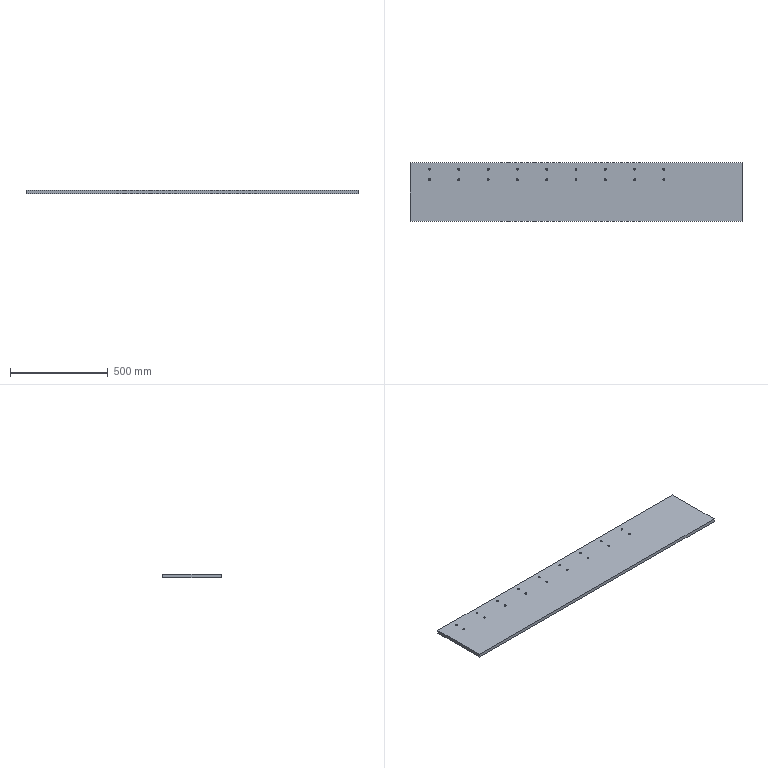Component | SolidWorks | X-AxisSlideMountingPlate-1 | 1 solid | 204 faces | box 1700 x 300 x 17 mm | volume 8657405 mm3 | cone 108 | cylinder 72 | plane 24 | commonest cylinder face diameters 5.5 x36 10 x36
build123d program:
from build123d import *

# Parameters (mm, degrees)
SKETCH1_W                                      = 1700
SKETCH1_H                                      = 300
BOSS_EXTRUDE1_DEPTH                            = 17
M5_HEX_SOCKET_HEAD_CAP_SCREW_CBORE1_AT_2_COUNT = 2
M5_HEX_SOCKET_HEAD_CAP_SCREW_CBORE1_AT_2_PITCH = 54
LPATTERN1_COUNT                                = 9
LPATTERN1_PITCH                                = 150


with BuildPart() as part:
    # Sketch1 → Boss-Extrude1 (new body)
    with BuildSketch(Plane.XY):
        Rectangle(SKETCH1_W, SKETCH1_H)
    extrude(amount=BOSS_EXTRUDE1_DEPTH)

    # Sketch3 → M5 Hex Socket Head Cap Screw CBORE1 (revolve, cut)
    with BuildSketch(Plane(origin=(450, 117, 17), x_dir=(0, -1, 0), z_dir=(1, 0, 0))):
        Polygon((0, 0), (0, 17), (2.775, 17), (2.75, 16.975), (2.75, 5.425), (2.775, 5.4), (5, 5.4), (5, 0.025), (5.025, 0), align=None)
    m5_hex_socket_head_cap_screw_cbore1 = revolve(axis=Axis((450, 117, 23.35), (0, 0, -1)), mode=Mode.SUBTRACT)

    # M5 Hex Socket Head Cap Screw CBORE1 at 2: M5 Hex Socket Head Cap Screw CBORE1 ×2
    with Locations(*[(0, -i * M5_HEX_SOCKET_HEAD_CAP_SCREW_CBORE1_AT_2_PITCH, 0) for i in range(1, M5_HEX_SOCKET_HEAD_CAP_SCREW_CBORE1_AT_2_COUNT)]):
        add(m5_hex_socket_head_cap_screw_cbore1, mode=Mode.SUBTRACT)

    # LPattern1: M5 Hex Socket Head Cap Screw CBORE1 ×9
    with Locations(*[(-i * LPATTERN1_PITCH, 0, 0) for i in range(1, LPATTERN1_COUNT)]):
        add(m5_hex_socket_head_cap_screw_cbore1, mode=Mode.SUBTRACT)

    # LPattern1 copy 1 sketch → LPattern1 copy 1 (revolve, cut)
    with BuildSketch(Plane(origin=(300, 63, 17), x_dir=(0, -1, 0), z_dir=(1, 0, 0))):
        Polygon((0, 0), (0, 17), (2.775, 17), (2.75, 16.975), (2.75, 5.425), (2.775, 5.4), (5, 5.4), (5, 0.025), (5.025, 0), align=None)
    revolve(axis=Axis((300, 63, 23.35), (0, 0, -1)), mode=Mode.SUBTRACT)

    # LPattern1 copy 2 sketch → LPattern1 copy 2 (revolve, cut)
    with BuildSketch(Plane(origin=(150, 63, 17), x_dir=(0, -1, 0), z_dir=(1, 0, 0))):
        Polygon((0, 0), (0, 17), (2.775, 17), (2.75, 16.975), (2.75, 5.425), (2.775, 5.4), (5, 5.4), (5, 0.025), (5.025, 0), align=None)
    revolve(axis=Axis((150, 63, 23.35), (0, 0, -1)), mode=Mode.SUBTRACT)

    # LPattern1 copy 3 sketch → LPattern1 copy 3 (revolve, cut)
    with BuildSketch(Plane(origin=(0, 63, 17), x_dir=(0, -1, 0), z_dir=(1, 0, 0))):
        Polygon((0, 0), (0, 17), (2.775, 17), (2.75, 16.975), (2.75, 5.425), (2.775, 5.4), (5, 5.4), (5, 0.025), (5.025, 0), align=None)
    revolve(axis=Axis((0, 63, 23.35), (0, 0, -1)), mode=Mode.SUBTRACT)

    # LPattern1 copy 4 sketch → LPattern1 copy 4 (revolve, cut)
    with BuildSketch(Plane(origin=(-150, 63, 17), x_dir=(0, -1, 0), z_dir=(1, 0, 0))):
        Polygon((0, 0), (0, 17), (2.775, 17), (2.75, 16.975), (2.75, 5.425), (2.775, 5.4), (5, 5.4), (5, 0.025), (5.025, 0), align=None)
    revolve(axis=Axis((-150, 63, 23.35), (0, 0, -1)), mode=Mode.SUBTRACT)

    # LPattern1 copy 5 sketch → LPattern1 copy 5 (revolve, cut)
    with BuildSketch(Plane(origin=(-300, 63, 17), x_dir=(0, -1, 0), z_dir=(1, 0, 0))):
        Polygon((0, 0), (0, 17), (2.775, 17), (2.75, 16.975), (2.75, 5.425), (2.775, 5.4), (5, 5.4), (5, 0.025), (5.025, 0), align=None)
    revolve(axis=Axis((-300, 63, 23.35), (0, 0, -1)), mode=Mode.SUBTRACT)

    # LPattern1 copy 6 sketch → LPattern1 copy 6 (revolve, cut)
    with BuildSketch(Plane(origin=(-450, 63, 17), x_dir=(0, -1, 0), z_dir=(1, 0, 0))):
        Polygon((0, 0), (0, 17), (2.775, 17), (2.75, 16.975), (2.75, 5.425), (2.775, 5.4), (5, 5.4), (5, 0.025), (5.025, 0), align=None)
    revolve(axis=Axis((-450, 63, 23.35), (0, 0, -1)), mode=Mode.SUBTRACT)

    # LPattern1 copy 7 sketch → LPattern1 copy 7 (revolve, cut)
    with BuildSketch(Plane(origin=(-600, 63, 17), x_dir=(0, -1, 0), z_dir=(1, 0, 0))):
        Polygon((0, 0), (0, 17), (2.775, 17), (2.75, 16.975), (2.75, 5.425), (2.775, 5.4), (5, 5.4), (5, 0.025), (5.025, 0), align=None)
    revolve(axis=Axis((-600, 63, 23.35), (0, 0, -1)), mode=Mode.SUBTRACT)

    # LPattern1 copy 8 sketch → LPattern1 copy 8 (revolve, cut)
    with BuildSketch(Plane(origin=(-750, 63, 17), x_dir=(0, -1, 0), z_dir=(1, 0, 0))):
        Polygon((0, 0), (0, 17), (2.775, 17), (2.75, 16.975), (2.75, 5.425), (2.775, 5.4), (5, 5.4), (5, 0.025), (5.025, 0), align=None)
    revolve(axis=Axis((-750, 63, 23.35), (0, 0, -1)), mode=Mode.SUBTRACT)


solid = part.part

# Placed as in the assembly
solid = solid.moved(Location((100, -90, 69), (0, 0, 0)))